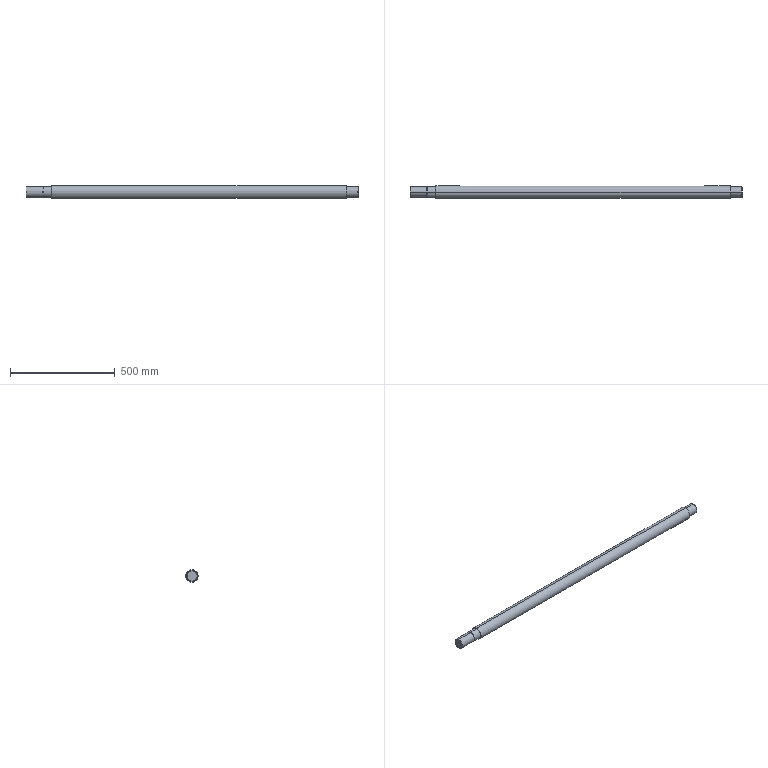Component | SolidWorks | DrivePulleyShaft-1 | 1 solid | 35 faces | volume 4197503 mm3 | cylinder 13 | cone 12 | plane 10 | commonest cylinder face diameters 50 x4 52 x3 60 x2 16 x2 18 x2